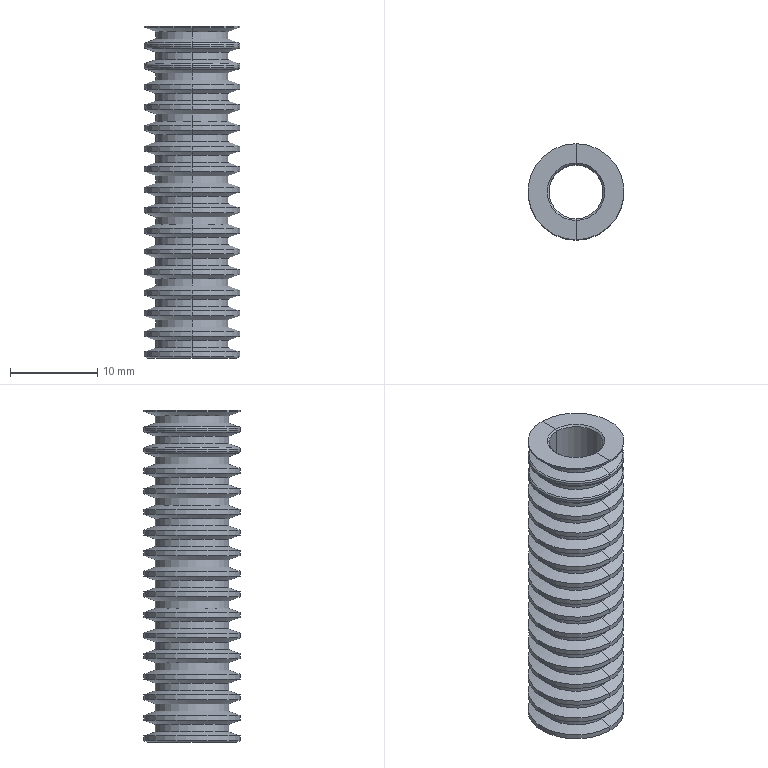Component | NX | DJZ_10_RACK_TRAVEL10 | 2 solids | 154 faces | volume 1610 mm3 | cone 70 | cylinder 68 | plane 8 | torus 8 | commonest cylinder face diameters 11 x34 8.4 x32 6.2 x2